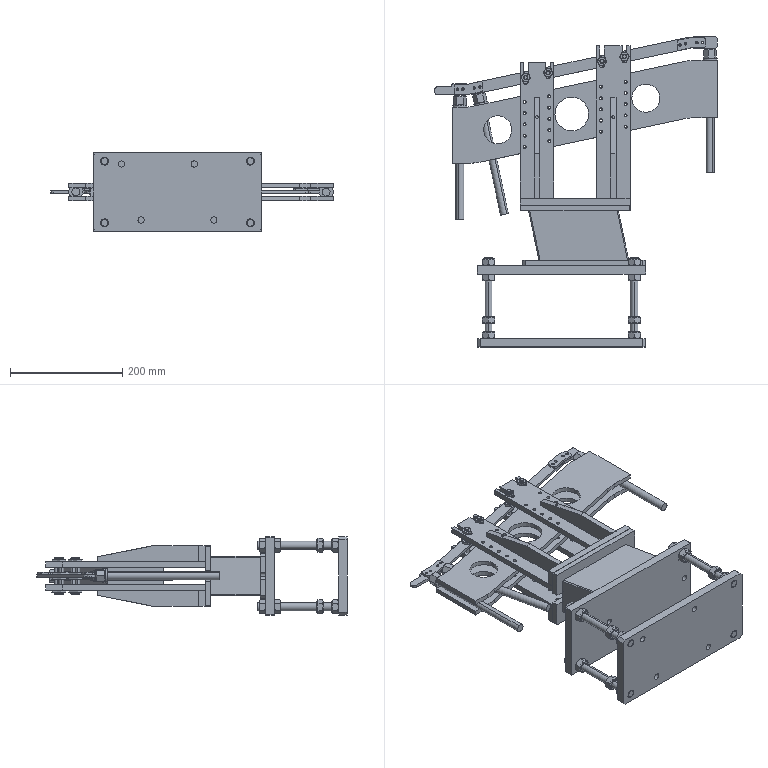Assembly | SolidWorks | mm | 64 component files | 64 solids | 1345 faces | box 503.26 x 553.16 x 140 mm | volume 4451689 mm3 | cylinder 569 | plane 562 | cone 214 | commonest cylinder face diameters 4.2 x80 5.5 x80 5 x56 11 x56 14 x54 8 x50 6.5 x48 8.5 x30
Bill of materials:
10AdjustmentPlate9.26 | 2 |  | Rectangular bar block with four obround slots through its wide side face and four small round holes in its narrow top face.
1Product25x2009.26 | 3 | AISI 1045 Steel, Cold Drawn | Long, slender cylindrical pin or rod with a hexagonal head and a thin flange collar at one end.
1VibrationTrackGuidePlate9.26 | 2 |  | Thin flat plate whose ends are offset (jogged), with three large round holes and four columns of small holes.
3RearBaffleConnectionPlate9.26 | 2 | AISI 1045 Steel, Cold Drawn | Flat plate with an angled (doglegged) outline, rounded corners and four round through holes.
3UpperBaffle9.26 | 1 | AISI 1045 Steel, Cold Drawn | Long, thin flat strip with rounded ends, four medium holes in the middle region and two small holes at each end.
3UpperBaffle-FrontSmallBaffle9.26 | 1 | AISI 1045 Steel, Cold Drawn | Flat plate with a stepped outline: a narrower arm and a wider end, rounded corners, and two round holes in the wider end.
3UpperBaffle-RearSmallBaffle9.26 | 1 | AISI 1045 Steel, Cold Drawn | Rectangular flat plate with rounded corners and two round through holes near one end.
4GuidePlateAdjustmentPlate9.26 | 1 | AISI 1045 Steel, Cold Drawn | Thin rectangular plate with an open-ended U-slot centered on each short edge.
5160#x98x70StraightVibrator9.26 | 1 | AISI 1045 Steel, Cold Drawn | Bracket-like part: a flat base plate with chamfered corners and a U-slot in each end, carrying a raised block with slanted (parallelogram-profile) side walls.
6GuidePlateG9.26 | 2 |  | Long rectangular flat plate with two open-ended slots at one end and many round holes in rows and a center line.
6GuidePlateH9.26 | 2 |  | Long rectangular flat plate with two open-ended slots at one end and a pattern of round holes, very similar to unnamed part.
M8Nut-29.26 | 16 | AISI 1045 Steel, Cold Drawn | Low-profile hexagonal nut-like part with a plain round center bore and chamfered corners on both faces.
UpperBaffleAdjustmentBolt9.26 | 4 |  | Solid straight cylindrical pin with a small chamfer at both ends; length roughly 7-8 times its diameter.
AdjustingScrew9.26 | 4 |  | Long, slender solid cylindrical rod with very small chamfers at both ends; length roughly 15-16 times its diameter.
AdjustmentFrameBasePlate9.26 | 1 | AISI 1045 Steel, Cold Drawn | Flat rectangular plate, about twice as long as it is wide, with four larger through holes near the corners and two smaller through holes on the lengthwise midline, one inboard of the left pair and one near the right edge.
LowerAdjustmentFrameBasePlate9.26 | 1 | AISI 1045 Steel, Cold Drawn | Flat rectangular plate, about twice as long as it is wide, with all four corners chamfered. It has four larger through holes near the corners and four smaller through holes in a staggered, non-symmetric pattern (two near the top edge, two near the bottom edge, offset sideways from each other).
M14Nut9.26 | 16 | AISI 1045 Steel, Cold Drawn | Elongated hexagonal prism with a central round through bore and chamfered/crowned ends. Length is roughly twice the across-flats width.
ReinforcingRib9.26 | 4 |  | Solid bar with a rectangular cross-section and constant width. Height is full over roughly the first 45% of the length, then tapers linearly to a lower height at the far end. One end face has a blind axial hole with a conical bottom, and a small transverse through hole runs through the height near the tapered end.
Mates:
1. coincident | 1VibrationTrackGuidePlate9.26-1 plane at (0, 0, 0) dir (0, 0, 1) | assembly plane at (0, 0, 0) dir (0, 0, 1)
2. coincident | 1VibrationTrackGuidePlate9.26-1 plane at (0, 0, 0) dir (0, 1, 0) | assembly plane at (0, 0, 0) dir (0, 1, 0)
3. coincident | 1VibrationTrackGuidePlate9.26-1 plane at (0, 0, 0) dir (1, 0, 0) | assembly plane at (0, 0, 0) dir (1, 0, 0)
4. distance | 1VibrationTrackGuidePlate9.26-1 face at (-4.204, 40, 8) dir (0, 0, 1) | 1VibrationTrackGuidePlate9.26-2 face at (-4.204, 40, 22.5) dir (0, 0, -1)
5. coincident | 1VibrationTrackGuidePlate9.26-1 face at (-30, 0, 8) dir (-1, 0, 0) | 1VibrationTrackGuidePlate9.26-2 face at (-30, 0, 30.5) dir (-1, 0, 0)
6. coincident | 1VibrationTrackGuidePlate9.26-1 face at (-30, -100, 0) dir (0, -1, 0) | 1VibrationTrackGuidePlate9.26-2 face at (-30, -100, 22.5) dir (0, -1, 0)
7. coincident | 1VibrationTrackGuidePlate9.26-1 face at (-4.204, 0, 8) dir (0, 1, 0) | 1Product25x2009.26-1 face at (-17.5, 0, 15.5) dir (0, -1, 0)
8. tangent | 1VibrationTrackGuidePlate9.26-2 face at (-4.204, 40, 22.5) dir (0, 0, -1) | 1Product25x2009.26-1 face at (-17.5, -200, 15.5) dir (0, 1, 0) r 7
9. tangent | 1VibrationTrackGuidePlate9.26-2 face at (-30, 0, 30.5) dir (-1, 0, 0) | 1Product25x2009.26-1 face at (-17.5, 3, 15.5) dir (0, -1, 0) r 12.5
10. coincident | 1VibrationTrackGuidePlate9.26-2 face at (4.112, 0.8741, 30.5) dir (-0.2079, 0.9781, 0) | 1Product25x2009.26-2 face at (20.435, 4.344, 15.5) dir (0.2079, -0.9781, 0)
11. tangent | 1VibrationTrackGuidePlate9.26-2 face at (-4.204, 40, 22.5) dir (0, 0, -1) | 1Product25x2009.26-2 face at (62.017, -191.286, 15.5) dir (-0.2079, 0.9781, 0) r 7
12. coincident | 1VibrationTrackGuidePlate9.26-2 face at (391.259, 83.165, 22.5) dir (0, 1, 0) | 1Product25x2009.26-3 face at (428.759, 83.165, 15) dir (0, -1, 0)
13. tangent | 1VibrationTrackGuidePlate9.26-1 face at (-4.204, 40, 8) dir (0, 0, 1) | 1Product25x2009.26-3 face at (428.759, -116.835, 15) dir (0, 1, 0) r 7
14. tangent | 1VibrationTrackGuidePlate9.26-1 face at (441.259, 83.165, 0) dir (1, 0, 0) | 1Product25x2009.26-3 face at (428.759, 86.165, 15) dir (0, -1, 0) r 12.5
15. coincident | 4GuidePlateAdjustmentPlate9.26-1 face at (112, -185, 69.5) dir (0, -1, 0) | 5160#x98x70StraightVibrator9.26-1 face at (265, -185, -19.75) dir (0, 1, 0)
16. distance | 4GuidePlateAdjustmentPlate9.26-1 face at (112, -175, 69.5) dir (0, 0, 1) | 5160#x98x70StraightVibrator9.26-1 face at (283.705, -273, 50.25) dir (0, 0, 1)
17. distance | 1VibrationTrackGuidePlate9.26-2 face at (-30, -100, 22.5) dir (0, -1, 0) | 5160#x98x70StraightVibrator9.26-1 face at (313.705, -283, 55.25) dir (0, -1, 0)
18. distance | 4GuidePlateAdjustmentPlate9.26-1 face at (90, -185, 5.25) dir (-1, 0, 0) | 5160#x98x70StraightVibrator9.26-1 edge at (105, -185, -17.75) dir (0, 0, 1)
19. coincident | 4GuidePlateAdjustmentPlate9.26-1 face at (112, -175, 69.5) dir (0, 1, 0) | 10AdjustmentPlate9.26-2 face at (90, -175, -10) dir (0, -1, 0)
20. distance | 1VibrationTrackGuidePlate9.26-2 face at (-4.204, 40, 30.5) dir (0, 0, 1) | 3UpperBaffle9.26-1 face at (-30, 41.665, 17.75) dir (0, 0, 1)
21. coincident | 10AdjustmentPlate9.26-2 face at (90, -163, -10) dir (0, 1, 0) | ReinforcingRib9.26-3 face at (261, -163, -39) dir (0, -1, 0)
22. coincident | 10AdjustmentPlate9.26-2 face at (90, -163, -10) dir (0, 1, 0) | ReinforcingRib9.26-3 face at (261, -163, -39) dir (0, -1, 0)
23. coincident | 10AdjustmentPlate9.26-2 face at (90, -163, -10) dir (0, 1, 0) | ReinforcingRib9.26-4 face at (125, -163, -39) dir (0, -1, 0)
24. coincident | 5160#x98x70StraightVibrator9.26-1 face at (313.705, -283, 55.25) dir (0, -1, 0) | AdjustmentFrameBasePlate9.26-1 face at (13.705, -283, -54.75) dir (0, 1, 0)
25. distance | 5160#x98x70StraightVibrator9.26-1 face at (313.705, -283, -24.75) dir (0, 0, -1) | AdjustmentFrameBasePlate9.26-1 face at (13.705, -298, -54.75) dir (0, 0, -1)
26. distance | 5160#x98x70StraightVibrator9.26-1 face at (93.705, -283, -24.75) dir (-1, 0, 0) | AdjustmentFrameBasePlate9.26-1 face at (13.705, -298, 85.25) dir (-1, 0, 0)
27. distance | LowerAdjustmentFrameBasePlate9.26-1 face at (13.705, -413, 85.25) dir (0, 1, 0) | AdjustmentFrameBasePlate9.26-1 face at (13.705, -298, -54.75) dir (0, -1, 0)
28. coincident | AdjustmentFrameBasePlate9.26-1 face at (13.705, -298, 85.25) dir (0, 0, 1) | LowerAdjustmentFrameBasePlate9.26-1 face at (13.705, -413, 85.25) dir (0, 0, 1)
29. coincident | AdjustmentFrameBasePlate9.26-1 face at (313.705, -298, 85.25) dir (1, 0, 0) | LowerAdjustmentFrameBasePlate9.26-1 face at (313.705, -413, -54.75) dir (1, 0, 0)
30. coincident | LowerAdjustmentFrameBasePlate9.26-1 axis at (293.705, -428, 70.25) dir (0, 1, 0) | AdjustingScrew9.26-1 axis at (293.705, -269, 70.25) dir (0, -1, 0)
31. coincident | LowerAdjustmentFrameBasePlate9.26-1 face at (13.705, -428, 85.25) dir (0, -1, 0) | AdjustingScrew9.26-1 face at (293.705, -428, 70.25) dir (0, -1, 0)
32. coincident | LowerAdjustmentFrameBasePlate9.26-1 axis at (293.705, -428, -39.75) dir (0, 1, 0) | AdjustingScrew9.26-2 axis at (293.705, -269, -39.75) dir (0, -1, 0)
33. coincident | LowerAdjustmentFrameBasePlate9.26-1 face at (13.705, -428, 85.25) dir (0, -1, 0) | AdjustingScrew9.26-2 face at (293.705, -428, -39.75) dir (0, -1, 0)
34. coincident | LowerAdjustmentFrameBasePlate9.26-1 axis at (33.705, -428, 70.25) dir (0, 1, 0) | AdjustingScrew9.26-3 axis at (33.705, -269, 70.25) dir (0, -1, 0)
35. coincident | LowerAdjustmentFrameBasePlate9.26-1 face at (13.705, -428, 85.25) dir (0, -1, 0) | AdjustingScrew9.26-3 face at (33.705, -428, 70.25) dir (0, -1, 0)
36. coincident | LowerAdjustmentFrameBasePlate9.26-1 axis at (33.705, -428, -39.75) dir (0, 1, 0) | AdjustingScrew9.26-4 axis at (33.705, -269, -39.75) dir (0, -1, 0)
37. coincident | LowerAdjustmentFrameBasePlate9.26-1 face at (13.705, -428, 85.25) dir (0, -1, 0) | AdjustingScrew9.26-4 face at (33.705, -428, -39.75) dir (0, -1, 0)
38. coincident | AdjustingScrew9.26-1 axis at (293.705, -269, 70.25) dir (0, -1, 0) | M14Nut9.26-1 axis at (293.705, -401, 70.25) dir (0, -1, 0)
39. coincident | LowerAdjustmentFrameBasePlate9.26-1 face at (13.705, -413, 85.25) dir (0, 1, 0) | M14Nut9.26-1 face at (304.811, -413, 64.086) dir (0, -1, 0)
40. coincident | 10AdjustmentPlate9.26-2 face at (286, -163, -10) dir (1, 0, 0) | 10AdjustmentPlate9.26-3 face at (286, -163, 40.5) dir (1, 0, 0)
41. coincident | ReinforcingRib9.26-1 face at (251, -163, 69.5) dir (0, -1, 0) | 10AdjustmentPlate9.26-3 face at (286, -163, 40.5) dir (0, 1, 0)
42. coincident | 10AdjustmentPlate9.26-3 axis at (132, -169, 58.5) dir (0, 0, -1) | 6GuidePlateG9.26-3 axis at (132, -169, 36.7) dir (0, 0, -1)
43. coincident | 10AdjustmentPlate9.26-3 axis at (108, -169, 58.5) dir (0, 0, -1) | 6GuidePlateG9.26-3 axis at (108, -169, 36.7) dir (0, 0, -1)
44. coincident | 10AdjustmentPlate9.26-3 face at (286, -175, 40.5) dir (0, 0, -1) | 6GuidePlateG9.26-3 face at (150, -175, 40.5) dir (0, 0, 1)
45. coincident | 10AdjustmentPlate9.26-3 axis at (244, -169, 58.5) dir (0, 0, -1) | 6GuidePlateH9.26-3 axis at (244, -169, 36.7) dir (0, 0, -1)
46. coincident | 10AdjustmentPlate9.26-3 axis at (268, -169, 58.5) dir (0, 0, -1) | 6GuidePlateH9.26-3 axis at (268, -169, 36.7) dir (0, 0, -1)
47. coincident | 10AdjustmentPlate9.26-3 face at (286, -175, 40.5) dir (0, 0, -1) | 6GuidePlateH9.26-3 face at (286, -175, 40.5) dir (0, 0, 1)
48. coincident | ReinforcingRib9.26-2 face at (114.958, -163, 69.5) dir (0, -1, 0) | 10AdjustmentPlate9.26-3 face at (286, -163, 40.5) dir (0, 1, 0)
49. coincident | 10AdjustmentPlate9.26-2 face at (90, -175, -10) dir (0, 0, 1) | 6GuidePlateG9.26-4 face at (150, -175, -10) dir (0, 0, -1)
50. coincident | 10AdjustmentPlate9.26-2 face at (90, -163, -10) dir (-1, 0, 0) | 6GuidePlateG9.26-4 face at (90, 80, -10) dir (-1, 0, 0)
51. coincident | 4GuidePlateAdjustmentPlate9.26-1 face at (112, -175, 69.5) dir (0, 1, 0) | 6GuidePlateG9.26-4 face at (150, -175, -10) dir (0, -1, 0)
52. coincident | 10AdjustmentPlate9.26-2 face at (90, -175, -10) dir (0, 0, 1) | 6GuidePlateH9.26-4 face at (286, -175, -10) dir (0, 0, -1)
53. coincident | 4GuidePlateAdjustmentPlate9.26-1 face at (112, -175, 69.5) dir (0, 1, 0) | 6GuidePlateH9.26-4 face at (286, -175, -10) dir (0, -1, 0)
54. coincident | 10AdjustmentPlate9.26-2 face at (286, -163, -10) dir (1, 0, 0) | 6GuidePlateH9.26-4 face at (286, 109, -10) dir (1, 0, 0)
55. coincident | 3UpperBaffle9.26-1 axis at (100, 52.697, 12.75) dir (0, 0, 1) | AdjustingBoltAssembly9.26-1/M8Nut-29.26-2 axis at (100, 52.697, 22.25) dir (0, 0, -1)
56. coincident | 6GuidePlateG9.26-4 face at (150, -175, -10) dir (0, 0, -1) | AdjustingBoltAssembly9.26-1/M8Nut-29.26-3 face at (108.66, 52.697, -10) dir (0, 0, 1)
57. coincident | 3UpperBaffle9.26-1 axis at (140, 61.199, 12.75) dir (0, 0, 1) | AdjustingBoltAssembly9.26-2/UpperBaffleAdjustmentBolt9.26-1 axis at (140, 61.199, 46.75) dir (0, 0, -1)
58. coincident | 6GuidePlateG9.26-3 face at (150, -175, 40.5) dir (0, 0, 1) | AdjustingBoltAssembly9.26-2/M8Nut-29.26-4 face at (148.528, 59.693, 40.5) dir (0, 0, -1)
59. coincident | 3UpperBaffle9.26-1 axis at (236, 81.605, 12.75) dir (0, 0, 1) | AdjustingBoltAssembly9.26-3/UpperBaffleAdjustmentBolt9.26-1 axis at (236, 81.605, 46.75) dir (0, 0, -1)
60. coincident | 6GuidePlateH9.26-3 face at (286, -175, 40.5) dir (0, 0, 1) | AdjustingBoltAssembly9.26-3/M8Nut-29.26-4 face at (244.528, 80.098, 40.5) dir (0, 0, -1)
61. coincident | 3UpperBaffle9.26-1 axis at (276, 90.107, 12.75) dir (0, 0, 1) | AdjustingBoltAssembly9.26-4/UpperBaffleAdjustmentBolt9.26-1 axis at (276, 90.107, 46.75) dir (0, 0, -1)
62. coincident | 6GuidePlateH9.26-3 face at (286, -175, 40.5) dir (0, 0, 1) | AdjustingBoltAssembly9.26-4/M8Nut-29.26-4 face at (284.613, 91.007, 40.5) dir (0, 0, -1)
63. distance | 3UpperBaffle9.26-1 face at (2.102, 21.665, 17.75) dir (0.2079, -0.9781, 0) | 1VibrationTrackGuidePlate9.26-2 face at (4.112, 0.8741, 30.5) dir (-0.2079, 0.9781, 0)
64. coincident | 3UpperBaffle9.26-1 face at (-30, 41.665, 17.75) dir (0, 0, 1) | 3UpperBaffle-RearSmallBaffle9.26-1 face at (-30, 41.165, 17.75) dir (0, 0, 1)
65. distance | 3UpperBaffle-RearSmallBaffle9.26-1 face at (397.291, 105.165, 17.75) dir (0, -1, 0) | 1Product25x2009.26-3 face at (420.712, 103.165, 6.719) dir (0, 1, 0)
66. coincident | 1VibrationTrackGuidePlate9.26-2 face at (441.259, 83.165, 22.5) dir (1, 0, 0) | 3UpperBaffle-RearSmallBaffle9.26-1 face at (441.259, 125.165, 17.75) dir (1, 0, 0)
67. coincident | 3UpperBaffle9.26-1 face at (-30, 41.665, 17.75) dir (0, 0, 1) | 3UpperBaffle-FrontSmallBaffle9.26-1 face at (-32, 42, 17.75) dir (0, 0, 1)
68. distance | 3UpperBaffle-FrontSmallBaffle9.26-1 face at (-32, 22, 17.75) dir (0, -1, 0) | 1Product25x2009.26-1 face at (-12.308, 20, 5.186) dir (0, 1, 0)
69. distance | 3UpperBaffle-FrontSmallBaffle9.26-1 face at (-62, 36, 17.75) dir (-1, 0, 0) | 1VibrationTrackGuidePlate9.26-2 face at (-30, 0, 30.5) dir (-1, 0, 0)
70. coincident | 3UpperBaffle-RearSmallBaffle9.26-1 face at (-30, 41.165, 17.75) dir (0, 0, 1) | 3RearBaffleConnectionPlate9.26-1 face at (370.259, 100.449, 17.75) dir (0, 0, -1)
71. distance | 3RearBaffleConnectionPlate9.26-1 face at (395.259, 124.165, 21.75) dir (0, 1, 0) | 3UpperBaffle-RearSmallBaffle9.26-1 face at (395.189, 125.165, 17.75) dir (0, 1, 0)
72. distance | 3RearBaffleConnectionPlate9.26-1 face at (420.259, 124.165, 21.75) dir (1, 0, 0) | 3UpperBaffle-RearSmallBaffle9.26-1 face at (441.259, 125.165, 17.75) dir (1, 0, 0)
73. coincident | 3UpperBaffle-FrontSmallBaffle9.26-1 face at (-32, 42, 17.75) dir (0, 0, 1) | 3RearBaffleConnectionPlate9.26-2 face at (23, 46.314, 17.75) dir (0, 0, -1)
74. distance | 3RearBaffleConnectionPlate9.26-2 face at (-27, 41, 21.75) dir (0, 1, 0) | 3UpperBaffle-FrontSmallBaffle9.26-1 face at (-32, 42, 17.75) dir (0, 1, 0)
75. distance | 3UpperBaffle-FrontSmallBaffle9.26-1 face at (-62, 36, 17.75) dir (-1, 0, 0) | 3RearBaffleConnectionPlate9.26-2 face at (-27, 22.598, 21.75) dir (-1, 0, 0)
76. coincident | UpperBaffleAdjustmentBolt9.26-1 plane at (0, 0, 0) dir (0, 0, 1) | AdjustingBoltAssembly9.26 plane at (0, 0, 0) dir (0, 0, 1)
77. coincident | UpperBaffleAdjustmentBolt9.26-1 plane at (0, 0, 0) dir (0, 1, 0) | AdjustingBoltAssembly9.26 plane at (0, 0, 0) dir (0, 1, 0)
78. coincident | UpperBaffleAdjustmentBolt9.26-1 plane at (0, 0, 0) dir (1, 0, 0) | AdjustingBoltAssembly9.26 plane at (0, 0, 0) dir (1, 0, 0)
79. coincident | UpperBaffleAdjustmentBolt9.26-1 axis at (0, 0, 64) dir (0, 0, -1) | M8Nut-29.26-1 axis at (0, 0, 30) dir (0, 0, -1)
80. coincident | UpperBaffleAdjustmentBolt9.26-1 axis at (0, 0, 64) dir (0, 0, -1) | M8Nut-29.26-2 axis at (0, 0, 39.5) dir (0, 0, -1)
81. distance | M8Nut-29.26-2 face at (8.66, 0, 35) dir (0, 0, -1) | M8Nut-29.26-1 face at (8.66, 0, 30) dir (0, 0, 1)
82. distance | M8Nut-29.26-2 face at (8.66, 0, 39.5) dir (0, 0, 1) | UpperBaffleAdjustmentBolt9.26-1 face at (0, 0, 65) dir (0, 0, 1)
83. coincident | UpperBaffleAdjustmentBolt9.26-1 axis at (0, 0, 64) dir (0, 0, -1) | M8Nut-29.26-3 axis at (0, 0, 7.25) dir (0, 0, -1)
84. coincident | UpperBaffleAdjustmentBolt9.26-1 axis at (0, 0, 64) dir (0, 0, -1) | M8Nut-29.26-4 axis at (0, 0, 62.25) dir (0, 0, -1)
85. distance | M8Nut-29.26-4 face at (8.528, -1.507, 57.75) dir (0, 0, -1) | M8Nut-29.26-3 face at (8.66, 0, 7.25) dir (0, 0, 1)
86. distance | UpperBaffleAdjustmentBolt9.26-1 face at (0, 0, 0) dir (0, 0, -1) | M8Nut-29.26-3 face at (8.66, 0, 2.75) dir (0, 0, -1)